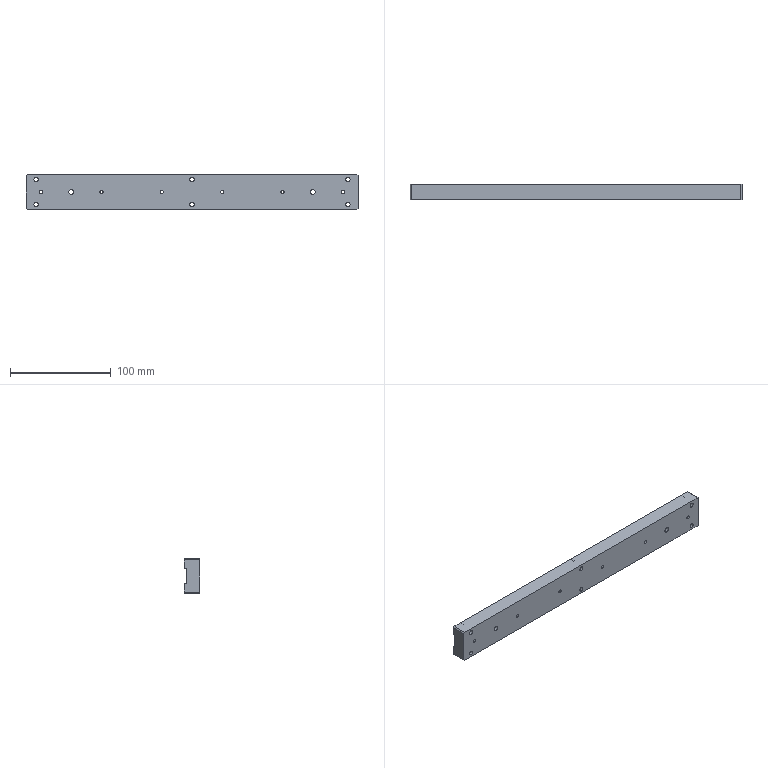Component | SolidWorks | A091-2 | 1 solid | 60 faces | box 330 x 15 x 34 mm | volume 154942 mm3 | cylinder 40 | plane 20 | commonest cylinder face diameters 8 x12 4.3 x12 3.3 x12 5 x4
build123d program:
from build123d import *

# Parameters (mm, degrees)
SKETCH1_W                                       = 34
SKETCH1_H                                       = 330
BOSS_EXTRUDE1_DEPTH                             = 15
SKETCH2_W                                       = 15
SKETCH2_H                                       = 330
CUT_EXTRUDE1_DEPTH                              = 2
CHAMFER1_SIZE                                   = 1
M4_TAPPED_HOLE1_D                               = 3.3
M4_HEX_SOCKET_HEAD_CAP_SCREW_CBORE1_D           = 4.3
M4_HEX_SOCKET_HEAD_CAP_SCREW_CBORE1_CBORE_D     = 8
M4_HEX_SOCKET_HEAD_CAP_SCREW_CBORE1_CBORE_DEPTH = 4.4
F_5_0_5_DIAMETER_HOLE1_D                        = 5


with BuildPart() as part:
    # Sketch1 → Boss-Extrude1 (new body)
    with BuildSketch(Plane.XY):
        Rectangle(SKETCH1_W, SKETCH1_H)
    extrude(amount=BOSS_EXTRUDE1_DEPTH)

    # Sketch2 → Cut-Extrude1 (cut)
    with BuildSketch(Plane.XY.offset(15)):
        Rectangle(SKETCH2_W, SKETCH2_H)
    extrude(amount=-CUT_EXTRUDE1_DEPTH, mode=Mode.SUBTRACT)

    # Chamfer1
    chamfer1_edges = [part.edges().sort_by_distance(p)[0] for p in [
        (17, -165, 7.5),
        (-17, -165, 7.5),
        (-17, 165, 7.5),
        (17, 165, 7.5),
    ]]
    chamfer(chamfer1_edges, length=CHAMFER1_SIZE)

    # M4 Tapped Hole1 (through all)
    with Locations(Plane.XY.offset(13)):
        with Locations((0, 150), (0, 90), (0, 30), (0, -30), (0, -90), (0, -150)):
            Hole(M4_TAPPED_HOLE1_D / 2)

    # M4 Hex Socket Head Cap Screw CBORE1 (through all)
    with Locations(Plane.XY.offset(15)):
        with Locations((12.5, 155), (-12.5, 155), (-12.5, -155), (12.5, -155), (-12.5, 0), (12.5, 0)):
            CounterBoreHole(M4_HEX_SOCKET_HEAD_CAP_SCREW_CBORE1_D / 2, M4_HEX_SOCKET_HEAD_CAP_SCREW_CBORE1_CBORE_D / 2, M4_HEX_SOCKET_HEAD_CAP_SCREW_CBORE1_CBORE_DEPTH)

    # 5.0 _5_ Diameter Hole1 (through all)
    with Locations(Plane.XY.offset(13)):
        with Locations((0, 120), (0, -120)):
            Hole(F_5_0_5_DIAMETER_HOLE1_D / 2)


solid = part.part

# Placed as in the assembly
solid = solid.moved(Location((150.381, 0, 83), (-90, 0, 90)))